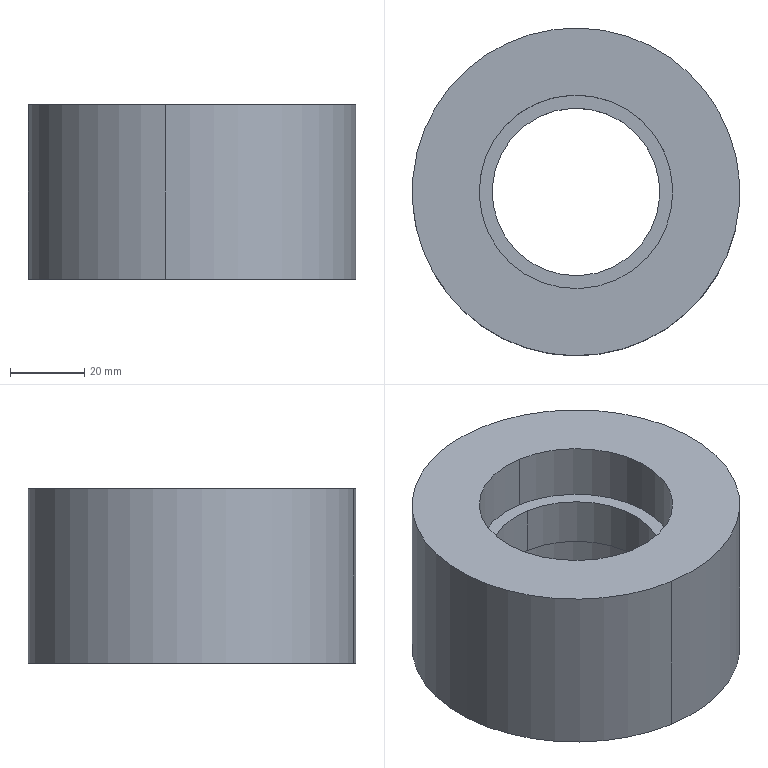Component | SolidWorks | NewTypeCurveBenderReinforcementPressingWheel-DoubleWheel-1 | 1 solid | 12 faces | box 88 x 88 x 47 mm | volume 192978 mm3 | cylinder 8 | plane 4 | commonest cylinder face diameters 52 x4 88 x2 45 x2
build123d program:
from build123d import *

# Parameters (mm, degrees)
SKETCH1_R           = 44
SKETCH1_R_2         = 22.5
BOSS_EXTRUDE1_DEPTH = 47
SKETCH2_R           = 26
CUT_EXTRUDE1_DEPTH  = 19
CUT_EXTRUDE2_START  = -15
SKETCH3_R           = 26
CUT_EXTRUDE2_DEPTH  = 15


with BuildPart() as part:
    # Sketch1 → Boss-Extrude1 (new body)
    with BuildSketch(Plane.XY):
        Circle(SKETCH1_R)
        Circle(SKETCH1_R_2, mode=Mode.SUBTRACT)
    extrude(amount=BOSS_EXTRUDE1_DEPTH)

    # Sketch2 → Cut-Extrude1 (cut)
    with BuildSketch(Plane(origin=(0, 0, 0), x_dir=(-1, 0, 0), z_dir=(0, 0, -1))):
        Circle(SKETCH2_R)
    extrude(amount=-CUT_EXTRUDE1_DEPTH, mode=Mode.SUBTRACT)

    # Sketch3 → Cut-Extrude2 (cut)
    with BuildSketch(Plane.XY.offset(47).offset(CUT_EXTRUDE2_START)):
        with Locations(Location((0, 0, 0), (0, 0, 180))):
            Circle(SKETCH3_R)
    extrude(amount=CUT_EXTRUDE2_DEPTH, mode=Mode.SUBTRACT)


solid = part.part

# Placed as in the assembly
solid = solid.moved(Location((-50, -201.632, -168), (0, 0, 0)))
STEP:
#1=COLOUR_RGB('',0.7922,0.8196,0.9333);
#2=FILL_AREA_STYLE_COLOUR('',#1);
#3=FILL_AREA_STYLE('',(#2));
#4=SURFACE_STYLE_FILL_AREA(#3);
#5=SURFACE_SIDE_STYLE('',(#4));
#6=SURFACE_STYLE_USAGE(.BOTH.,#5);
#7=PRESENTATION_STYLE_ASSIGNMENT((#6));
#8=CARTESIAN_POINT('',(-2.136,-8.948,-5.354));
#9=VERTEX_POINT('',#8);
#10=CARTESIAN_POINT('',(-1.801,-6.928,-5.354));
#11=VERTEX_POINT('',#10);
#12=CARTESIAN_POINT('',(-1.969,-7.938,-5.354));
#13=DIRECTION('',(-0.,0.,1.));
#14=DIRECTION('',(0.1639,0.9865,0.));
#15=AXIS2_PLACEMENT_3D('',#12,#13,#14);
#16=CIRCLE('',#15,1.024);
#17=EDGE_CURVE('',#9,#11,#16,.T.);
#18=ORIENTED_EDGE('',*,*,#17,.F.);
#19=CARTESIAN_POINT('',(-2.136,-8.948,-4.764));
#20=VERTEX_POINT('',#19);
#21=CARTESIAN_POINT('',(-2.136,-8.948,-5.354));
#22=DIRECTION('',(-0.,0.,1.));
#23=VECTOR('',#22,39.37);
#24=LINE('',#21,#23);
#25=EDGE_CURVE('',#9,#20,#24,.T.);
#26=ORIENTED_EDGE('',*,*,#25,.T.);
#27=CARTESIAN_POINT('',(-1.801,-6.928,-4.764));
#28=VERTEX_POINT('',#27);
#29=CARTESIAN_POINT('',(-1.969,-7.938,-4.764));
#30=DIRECTION('',(-0.,0.,1.));
#31=DIRECTION('',(0.1639,0.9865,0.));
#32=AXIS2_PLACEMENT_3D('',#29,#30,#31);
#33=CIRCLE('',#32,1.024);
#34=EDGE_CURVE('',#20,#28,#33,.T.);
#35=ORIENTED_EDGE('',*,*,#34,.T.);
#36=CARTESIAN_POINT('',(-1.801,-6.928,-5.354));
#37=DIRECTION('',(-0.,0.,1.));
#38=VECTOR('',#37,39.37);
#39=LINE('',#36,#38);
#40=EDGE_CURVE('',#11,#28,#39,.T.);
#41=ORIENTED_EDGE('',*,*,#40,.F.);
#42=EDGE_LOOP('',(#18,#26,#35,#41));
#43=FACE_OUTER_BOUND('',#42,.T.);
#44=CARTESIAN_POINT('',(-1.969,-7.938,-5.354));
#45=DIRECTION('',(-0.,0.,1.));
#46=DIRECTION('',(0.1639,0.9865,0.));
#47=AXIS2_PLACEMENT_3D('',#44,#45,#46);
#48=CYLINDRICAL_SURFACE('',#47,1.024);
#49=ADVANCED_FACE('',(#43),#48,.F.);
#50=CARTESIAN_POINT('',(-1.801,-6.928,-5.866));
#51=VERTEX_POINT('',#50);
#52=CARTESIAN_POINT('',(-2.136,-8.948,-5.866));
#53=VERTEX_POINT('',#52);
#54=CARTESIAN_POINT('',(-1.969,-7.938,-5.866));
#55=DIRECTION('',(0.,-0.,-1.));
#56=DIRECTION('',(-0.1639,-0.9865,0.));
#57=AXIS2_PLACEMENT_3D('',#54,#55,#56);
#58=CIRCLE('',#57,1.024);
#59=EDGE_CURVE('',#51,#53,#58,.T.);
#60=ORIENTED_EDGE('',*,*,#59,.F.);
#61=CARTESIAN_POINT('',(-1.801,-6.928,-6.614));
#62=VERTEX_POINT('',#61);
#63=CARTESIAN_POINT('',(-1.801,-6.928,-5.866));
#64=DIRECTION('',(0.,-0.,-1.));
#65=VECTOR('',#64,39.37);
#66=LINE('',#63,#65);
#67=EDGE_CURVE('',#51,#62,#66,.T.);
#68=ORIENTED_EDGE('',*,*,#67,.T.);
#69=CARTESIAN_POINT('',(-2.136,-8.948,-6.614));
#70=VERTEX_POINT('',#69);
#71=CARTESIAN_POINT('',(-1.969,-7.938,-6.614));
#72=DIRECTION('',(0.,-0.,-1.));
#73=DIRECTION('',(-0.1639,-0.9865,0.));
#74=AXIS2_PLACEMENT_3D('',#71,#72,#73);
#75=CIRCLE('',#74,1.024);
#76=EDGE_CURVE('',#62,#70,#75,.T.);
#77=ORIENTED_EDGE('',*,*,#76,.T.);
#78=CARTESIAN_POINT('',(-2.136,-8.948,-5.866));
#79=DIRECTION('',(0.,-0.,-1.));
#80=VECTOR('',#79,39.37);
#81=LINE('',#78,#80);
#82=EDGE_CURVE('',#53,#70,#81,.T.);
#83=ORIENTED_EDGE('',*,*,#82,.F.);
#84=EDGE_LOOP('',(#60,#68,#77,#83));
#85=FACE_OUTER_BOUND('',#84,.T.);
#86=CARTESIAN_POINT('',(-1.969,-7.938,-5.866));
#87=DIRECTION('',(0.,-0.,-1.));
#88=DIRECTION('',(-0.1639,-0.9865,0.));
#89=AXIS2_PLACEMENT_3D('',#86,#87,#88);
#90=CYLINDRICAL_SURFACE('',#89,1.024);
#91=ADVANCED_FACE('',(#85),#90,.F.);
#92=CARTESIAN_POINT('',(-1.685,-6.229,-4.764));
#93=VERTEX_POINT('',#92);
#94=CARTESIAN_POINT('',(-2.252,-9.647,-4.764));
#95=VERTEX_POINT('',#94);
#96=CARTESIAN_POINT('',(-1.969,-7.938,-4.764));
#97=DIRECTION('',(-0.,0.,1.));
#98=DIRECTION('',(0.1639,0.9865,0.));
#99=AXIS2_PLACEMENT_3D('',#96,#97,#98);
#100=CIRCLE('',#99,1.732);
#101=EDGE_CURVE('',#93,#95,#100,.T.);
#102=ORIENTED_EDGE('',*,*,#101,.F.);
#103=CARTESIAN_POINT('',(-1.685,-6.229,-6.614));
#104=VERTEX_POINT('',#103);
#105=CARTESIAN_POINT('',(-1.685,-6.229,-4.764));
#106=DIRECTION('',(0.,-0.,-1.));
#107=VECTOR('',#106,39.37);
#108=LINE('',#105,#107);
#109=EDGE_CURVE('',#93,#104,#108,.T.);
#110=ORIENTED_EDGE('',*,*,#109,.T.);
#111=CARTESIAN_POINT('',(-2.252,-9.647,-6.614));
#112=VERTEX_POINT('',#111);
#113=CARTESIAN_POINT('',(-1.969,-7.938,-6.614));
#114=DIRECTION('',(-0.,0.,1.));
#115=DIRECTION('',(0.1639,0.9865,0.));
#116=AXIS2_PLACEMENT_3D('',#113,#114,#115);
#117=CIRCLE('',#116,1.732);
#118=EDGE_CURVE('',#104,#112,#117,.T.);
#119=ORIENTED_EDGE('',*,*,#118,.T.);
#120=CARTESIAN_POINT('',(-2.252,-9.647,-4.764));
#121=DIRECTION('',(0.,-0.,-1.));
#122=VECTOR('',#121,39.37);
#123=LINE('',#120,#122);
#124=EDGE_CURVE('',#95,#112,#123,.T.);
#125=ORIENTED_EDGE('',*,*,#124,.F.);
#126=EDGE_LOOP('',(#102,#110,#119,#125));
#127=FACE_OUTER_BOUND('',#126,.T.);
#128=CARTESIAN_POINT('',(-1.969,-7.938,-4.764));
#129=DIRECTION('',(0.,-0.,-1.));
#130=DIRECTION('',(-0.1639,-0.9865,0.));
#131=AXIS2_PLACEMENT_3D('',#128,#129,#130);
#132=CYLINDRICAL_SURFACE('',#131,1.732);
#133=ADVANCED_FACE('',(#127),#132,.T.);
#134=CARTESIAN_POINT('',(-2.114,-8.812,-5.354));
#135=VERTEX_POINT('',#134);
#136=CARTESIAN_POINT('',(-1.823,-7.064,-5.354));
#137=VERTEX_POINT('',#136);
#138=CARTESIAN_POINT('',(-1.969,-7.938,-5.354));
#139=DIRECTION('',(-0.,0.,1.));
#140=DIRECTION('',(0.1639,0.9865,0.));
#141=AXIS2_PLACEMENT_3D('',#138,#139,#140);
#142=CIRCLE('',#141,0.8858);
#143=EDGE_CURVE('',#135,#137,#142,.T.);
#144=ORIENTED_EDGE('',*,*,#143,.T.);
#145=CARTESIAN_POINT('',(-1.823,-7.064,-5.866));
#146=VERTEX_POINT('',#145);
#147=CARTESIAN_POINT('',(-1.823,-7.064,-4.764));
#148=DIRECTION('',(0.,-0.,-1.));
#149=VECTOR('',#148,39.37);
#150=LINE('',#147,#149);
#151=EDGE_CURVE('',#137,#146,#150,.T.);
#152=ORIENTED_EDGE('',*,*,#151,.T.);
#153=CARTESIAN_POINT('',(-2.114,-8.812,-5.866));
#154=VERTEX_POINT('',#153);
#155=CARTESIAN_POINT('',(-1.969,-7.938,-5.866));
#156=DIRECTION('',(0.,-0.,-1.));
#157=DIRECTION('',(-0.1639,-0.9865,0.));
#158=AXIS2_PLACEMENT_3D('',#155,#156,#157);
#159=CIRCLE('',#158,0.8858);
#160=EDGE_CURVE('',#146,#154,#159,.T.);
#161=ORIENTED_EDGE('',*,*,#160,.T.);
#162=CARTESIAN_POINT('',(-2.114,-8.812,-4.764));
#163=DIRECTION('',(0.,-0.,-1.));
#164=VECTOR('',#163,39.37);
#165=LINE('',#162,#164);
#166=EDGE_CURVE('',#135,#154,#165,.T.);
#167=ORIENTED_EDGE('',*,*,#166,.F.);
#168=EDGE_LOOP('',(#144,#152,#161,#167));
#169=FACE_OUTER_BOUND('',#168,.T.);
#170=CARTESIAN_POINT('',(-1.969,-7.938,-4.764));
#171=DIRECTION('',(0.,-0.,-1.));
#172=DIRECTION('',(-0.1639,-0.9865,0.));
#173=AXIS2_PLACEMENT_3D('',#170,#171,#172);
#174=CYLINDRICAL_SURFACE('',#173,0.8858);
#175=ADVANCED_FACE('',(#169),#174,.F.);
#176=ORIENTED_EDGE('',*,*,#151,.F.);
#177=CARTESIAN_POINT('',(-1.969,-7.938,-5.354));
#178=DIRECTION('',(-0.,0.,1.));
#179=DIRECTION('',(0.1639,0.9865,0.));
#180=AXIS2_PLACEMENT_3D('',#177,#178,#179);
#181=CIRCLE('',#180,0.8858);
#182=EDGE_CURVE('',#137,#135,#181,.T.);
#183=ORIENTED_EDGE('',*,*,#182,.T.);
#184=ORIENTED_EDGE('',*,*,#166,.T.);
#185=CARTESIAN_POINT('',(-1.969,-7.938,-5.866));
#186=DIRECTION('',(0.,-0.,-1.));
#187=DIRECTION('',(-0.1639,-0.9865,0.));
#188=AXIS2_PLACEMENT_3D('',#185,#186,#187);
#189=CIRCLE('',#188,0.8858);
#190=EDGE_CURVE('',#154,#146,#189,.T.);
#191=ORIENTED_EDGE('',*,*,#190,.T.);
#192=EDGE_LOOP('',(#176,#183,#184,#191));
#193=FACE_OUTER_BOUND('',#192,.T.);
#194=CARTESIAN_POINT('',(-1.969,-7.938,-4.764));
#195=DIRECTION('',(0.,-0.,-1.));
#196=DIRECTION('',(-0.1639,-0.9865,0.));
#197=AXIS2_PLACEMENT_3D('',#194,#195,#196);
#198=CYLINDRICAL_SURFACE('',#197,0.8858);
#199=ADVANCED_FACE('',(#193),#198,.F.);
#200=CARTESIAN_POINT('',(-1.969,-7.938,-4.764));
#201=DIRECTION('',(-0.,0.,1.));
#202=DIRECTION('',(0.1639,0.9865,0.));
#203=AXIS2_PLACEMENT_3D('',#200,#201,#202);
#204=CIRCLE('',#203,1.024);
#205=EDGE_CURVE('',#28,#20,#204,.T.);
#206=ORIENTED_EDGE('',*,*,#205,.F.);
#207=ORIENTED_EDGE('',*,*,#34,.F.);
#208=EDGE_LOOP('',(#206,#207));
#209=FACE_BOUND('',#208,.T.);
#210=CARTESIAN_POINT('',(-1.969,-7.938,-4.764));
#211=DIRECTION('',(-0.,0.,1.));
#212=DIRECTION('',(0.1639,0.9865,0.));
#213=AXIS2_PLACEMENT_3D('',#210,#211,#212);
#214=CIRCLE('',#213,1.732);
#215=EDGE_CURVE('',#95,#93,#214,.T.);
#216=ORIENTED_EDGE('',*,*,#215,.T.);
#217=ORIENTED_EDGE('',*,*,#101,.T.);
#218=EDGE_LOOP('',(#216,#217));
#219=FACE_OUTER_BOUND('',#218,.T.);
#220=CARTESIAN_POINT('',(-1.969,-7.938,-4.764));
#221=DIRECTION('',(-0.,0.,1.));
#222=DIRECTION('',(0.1639,0.9865,0.));
#223=AXIS2_PLACEMENT_3D('',#220,#221,#222);
#224=PLANE('',#223);
#225=ADVANCED_FACE('',(#209,#219),#224,.T.);
#226=CARTESIAN_POINT('',(-1.969,-7.938,-6.614));
#227=DIRECTION('',(0.,-0.,-1.));
#228=DIRECTION('',(-0.1639,-0.9865,0.));
#229=AXIS2_PLACEMENT_3D('',#226,#227,#228);
#230=CIRCLE('',#229,1.024);
#231=EDGE_CURVE('',#70,#62,#230,.T.);
#232=ORIENTED_EDGE('',*,*,#231,.F.);
#233=ORIENTED_EDGE('',*,*,#76,.F.);
#234=EDGE_LOOP('',(#232,#233));
#235=FACE_BOUND('',#234,.T.);
#236=CARTESIAN_POINT('',(-1.969,-7.938,-6.614));
#237=DIRECTION('',(-0.,0.,1.));
#238=DIRECTION('',(0.1639,0.9865,0.));
#239=AXIS2_PLACEMENT_3D('',#236,#237,#238);
#240=CIRCLE('',#239,1.732);
#241=EDGE_CURVE('',#112,#104,#240,.T.);
#242=ORIENTED_EDGE('',*,*,#241,.F.);
#243=ORIENTED_EDGE('',*,*,#118,.F.);
#244=EDGE_LOOP('',(#242,#243));
#245=FACE_OUTER_BOUND('',#244,.T.);
#246=CARTESIAN_POINT('',(-1.969,-7.938,-6.614));
#247=DIRECTION('',(-0.,0.,1.));
#248=DIRECTION('',(0.1639,0.9865,0.));
#249=AXIS2_PLACEMENT_3D('',#246,#247,#248);
#250=PLANE('',#249);
#251=ADVANCED_FACE('',(#235,#245),#250,.F.);
#252=ORIENTED_EDGE('',*,*,#109,.F.);
#253=ORIENTED_EDGE('',*,*,#215,.F.);
#254=ORIENTED_EDGE('',*,*,#124,.T.);
#255=ORIENTED_EDGE('',*,*,#241,.T.);
#256=EDGE_LOOP('',(#252,#253,#254,#255));
#257=FACE_OUTER_BOUND('',#256,.T.);
#258=CARTESIAN_POINT('',(-1.969,-7.938,-4.764));
#259=DIRECTION('',(0.,-0.,-1.));
#260=DIRECTION('',(-0.1639,-0.9865,0.));
#261=AXIS2_PLACEMENT_3D('',#258,#259,#260);
#262=CYLINDRICAL_SURFACE('',#261,1.732);
#263=ADVANCED_FACE('',(#257),#262,.T.);
#264=ORIENTED_EDGE('',*,*,#67,.F.);
#265=CARTESIAN_POINT('',(-1.969,-7.938,-5.866));
#266=DIRECTION('',(0.,-0.,-1.));
#267=DIRECTION('',(-0.1639,-0.9865,0.));
#268=AXIS2_PLACEMENT_3D('',#265,#266,#267);
#269=CIRCLE('',#268,1.024);
#270=EDGE_CURVE('',#53,#51,#269,.T.);
#271=ORIENTED_EDGE('',*,*,#270,.F.);
#272=ORIENTED_EDGE('',*,*,#82,.T.);
#273=ORIENTED_EDGE('',*,*,#231,.T.);
#274=EDGE_LOOP('',(#264,#271,#272,#273));
#275=FACE_OUTER_BOUND('',#274,.T.);
#276=CARTESIAN_POINT('',(-1.969,-7.938,-5.866));
#277=DIRECTION('',(0.,-0.,-1.));
#278=DIRECTION('',(-0.1639,-0.9865,0.));
#279=AXIS2_PLACEMENT_3D('',#276,#277,#278);
#280=CYLINDRICAL_SURFACE('',#279,1.024);
#281=ADVANCED_FACE('',(#275),#280,.F.);
#282=ORIENTED_EDGE('',*,*,#190,.F.);
#283=ORIENTED_EDGE('',*,*,#160,.F.);
#284=EDGE_LOOP('',(#282,#283));
#285=FACE_BOUND('',#284,.T.);
#286=ORIENTED_EDGE('',*,*,#270,.T.);
#287=ORIENTED_EDGE('',*,*,#59,.T.);
#288=EDGE_LOOP('',(#286,#287));
#289=FACE_OUTER_BOUND('',#288,.T.);
#290=CARTESIAN_POINT('',(-1.969,-7.938,-5.866));
#291=DIRECTION('',(0.,-0.,-1.));
#292=DIRECTION('',(-0.1639,-0.9865,-0.));
#293=AXIS2_PLACEMENT_3D('',#290,#291,#292);
#294=PLANE('',#293);
#295=ADVANCED_FACE('',(#285,#289),#294,.T.);
#296=ORIENTED_EDGE('',*,*,#25,.F.);
#297=CARTESIAN_POINT('',(-1.969,-7.938,-5.354));
#298=DIRECTION('',(-0.,0.,1.));
#299=DIRECTION('',(0.1639,0.9865,0.));
#300=AXIS2_PLACEMENT_3D('',#297,#298,#299);
#301=CIRCLE('',#300,1.024);
#302=EDGE_CURVE('',#11,#9,#301,.T.);
#303=ORIENTED_EDGE('',*,*,#302,.F.);
#304=ORIENTED_EDGE('',*,*,#40,.T.);
#305=ORIENTED_EDGE('',*,*,#205,.T.);
#306=EDGE_LOOP('',(#296,#303,#304,#305));
#307=FACE_OUTER_BOUND('',#306,.T.);
#308=CARTESIAN_POINT('',(-1.969,-7.938,-5.354));
#309=DIRECTION('',(-0.,0.,1.));
#310=DIRECTION('',(0.1639,0.9865,0.));
#311=AXIS2_PLACEMENT_3D('',#308,#309,#310);
#312=CYLINDRICAL_SURFACE('',#311,1.024);
#313=ADVANCED_FACE('',(#307),#312,.F.);
#314=ORIENTED_EDGE('',*,*,#143,.F.);
#315=ORIENTED_EDGE('',*,*,#182,.F.);
#316=EDGE_LOOP('',(#314,#315));
#317=FACE_BOUND('',#316,.T.);
#318=ORIENTED_EDGE('',*,*,#302,.T.);
#319=ORIENTED_EDGE('',*,*,#17,.T.);
#320=EDGE_LOOP('',(#318,#319));
#321=FACE_OUTER_BOUND('',#320,.T.);
#322=CARTESIAN_POINT('',(-1.969,-7.938,-5.354));
#323=DIRECTION('',(-0.,0.,1.));
#324=DIRECTION('',(0.1639,0.9865,0.));
#325=AXIS2_PLACEMENT_3D('',#322,#323,#324);
#326=PLANE('',#325);
#327=ADVANCED_FACE('',(#317,#321),#326,.T.);
#328=CLOSED_SHELL('',(#49,#91,#133,#175,#199,#225,#251,#263,#281,#295,#313,#327));
#329=MANIFOLD_SOLID_BREP('',#328);
#330=STYLED_ITEM('',(#7),#329);
#331=PRESENTATION_LAYER_ASSIGNMENT('','',(#330));
#332=(LENGTH_UNIT()NAMED_UNIT(*)SI_UNIT($,.METRE.));
#333=LENGTH_MEASURE_WITH_UNIT(LENGTH_MEASURE(0.0254),#332);
#334=DIMENSIONAL_EXPONENTS(1.,0.,0.,0.,0.,0.,0.);
#335=(CONVERSION_BASED_UNIT('',#333)LENGTH_UNIT()NAMED_UNIT(#334));
#336=UNCERTAINTY_MEASURE_WITH_UNIT(LENGTH_MEASURE(0.00001),#335,'','');
#337=(NAMED_UNIT(*)PLANE_ANGLE_UNIT()SI_UNIT($,.RADIAN.));
#338=(NAMED_UNIT(*)SI_UNIT($,.STERADIAN.)SOLID_ANGLE_UNIT());
#339=(GEOMETRIC_REPRESENTATION_CONTEXT(3)GLOBAL_UNCERTAINTY_ASSIGNED_CONTEXT((#336))GLOBAL_UNIT_ASSIGNED_CONTEXT((#335,#337,#338))REPRESENTATION_CONTEXT('',''));
#340=MECHANICAL_DESIGN_GEOMETRIC_PRESENTATION_REPRESENTATION('',(#330),#339);
#341=CARTESIAN_POINT('',(0.,0.,0.));
#342=DIRECTION('',(0.,0.,1.));
#343=DIRECTION('',(1.,0.,0.));
#344=AXIS2_PLACEMENT_3D('',#341,#342,#343);
#345=(LENGTH_UNIT()NAMED_UNIT(*)SI_UNIT($,.METRE.));
#346=LENGTH_MEASURE_WITH_UNIT(LENGTH_MEASURE(0.0254),#345);
#347=DIMENSIONAL_EXPONENTS(1.,0.,0.,0.,0.,0.,0.);
#348=(CONVERSION_BASED_UNIT('',#346)LENGTH_UNIT()NAMED_UNIT(#347));
#349=UNCERTAINTY_MEASURE_WITH_UNIT(LENGTH_MEASURE(0.00001),#348,'','');
#350=(NAMED_UNIT(*)PLANE_ANGLE_UNIT()SI_UNIT($,.RADIAN.));
#351=(NAMED_UNIT(*)SI_UNIT($,.STERADIAN.)SOLID_ANGLE_UNIT());
#352=(GEOMETRIC_REPRESENTATION_CONTEXT(3)GLOBAL_UNCERTAINTY_ASSIGNED_CONTEXT((#349))GLOBAL_UNIT_ASSIGNED_CONTEXT((#348,#350,#351))REPRESENTATION_CONTEXT('',''));
#353=ADVANCED_BREP_SHAPE_REPRESENTATION('',(#329,#344),#352);